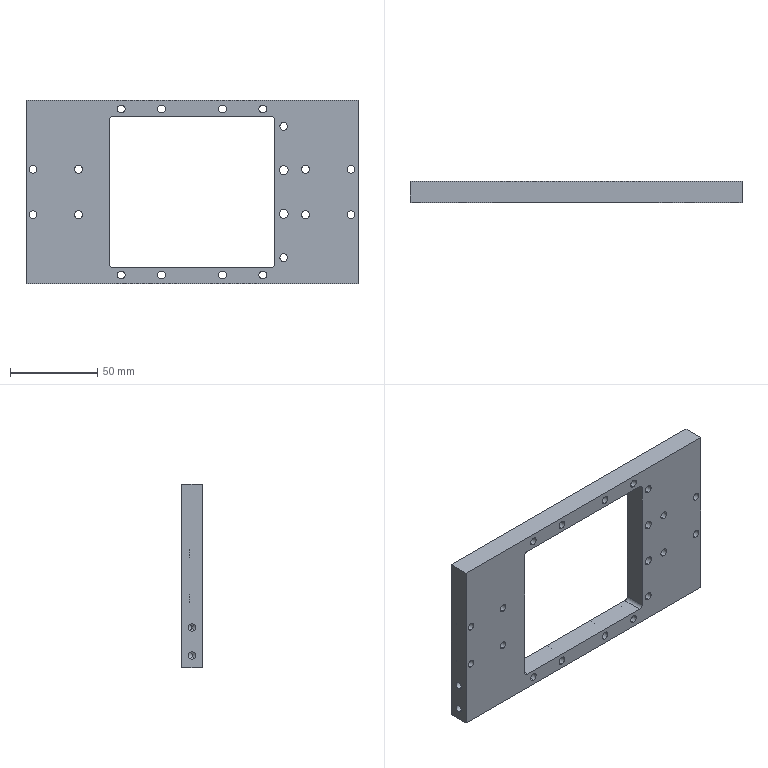Component | SolidWorks | 05-1 | 1 solid | 116 faces | box 190 x 12 x 105 mm | volume 134418 mm3 | cylinder 84 | plane 28 | cone 4 | commonest cylinder face diameters 4.5 x36 8 x20 7.9 x16 4.2 x4 5 x4 4 x4
build123d program:
from build123d import *

# Parameters (mm, degrees)
SKETCH1_W                                       = 190
SKETCH1_H                                       = 105
EXTRUDE1_DEPTH                                  = 6
SKETCH4_W                                       = 95
SKETCH4_H                                       = 86
CUT_EXTRUDE2_DEPTH                              = 110.203
M4_HEX_SOCKET_HEAD_CAP_SCREW_CBORE4_D           = 4.5
M4_HEX_SOCKET_HEAD_CAP_SCREW_CBORE4_CBORE_D     = 7.9
M4_HEX_SOCKET_HEAD_CAP_SCREW_CBORE4_CBORE_DEPTH = 4.4
FILLET1_R                                       = 2
M4_HEX_SOCKET_HEAD_CAP_SCREW_CBORE5_D           = 4.5
M4_HEX_SOCKET_HEAD_CAP_SCREW_CBORE5_CBORE_D     = 8
M4_HEX_SOCKET_HEAD_CAP_SCREW_CBORE5_CBORE_DEPTH = 4.4
SKETCH12_R                                      = 2.5
CUT_EXTRUDE1_DEPTH                              = 35
M5_TAPPED_HOLE1_D                               = 4.2
M5_TAPPED_HOLE1_DEPTH                           = 14
M5_TAPPED_HOLE1_TIP                             = 1.262


with BuildPart() as part:
    # Sketch1 → Extrude1 (new, symmetric)
    with BuildSketch(Plane(origin=(0, 0, 0), x_dir=(1, 0, 0), z_dir=(0, 1, 0))):
        Rectangle(SKETCH1_W, SKETCH1_H)
    extrude(amount=EXTRUDE1_DEPTH, both=True)

    # Sketch4 → Cut-Extrude2 (cut, through all)
    with BuildSketch(Plane(origin=(0, 6, 0), x_dir=(1, 0, 0), z_dir=(0, 1, 0))):
        Rectangle(SKETCH4_W, SKETCH4_H)
    extrude(amount=-CUT_EXTRUDE2_DEPTH, mode=Mode.SUBTRACT)

    # M4 Hex Socket Head Cap Screw CBORE4 (through all)
    with Locations(Plane(origin=(0, 6, 0), x_dir=(1, 0, 0), z_dir=(0, 1, 0))):
        with Locations((91, -13), (65, -13), (91, 13), (65, 13), (-65, -13), (-91, -13), (-65, 13), (-91, 13)):
            CounterBoreHole(M4_HEX_SOCKET_HEAD_CAP_SCREW_CBORE4_D / 2, M4_HEX_SOCKET_HEAD_CAP_SCREW_CBORE4_CBORE_D / 2, M4_HEX_SOCKET_HEAD_CAP_SCREW_CBORE4_CBORE_DEPTH)

    # Fillet1
    fillet1_edges = [part.edges().sort_by_distance(p)[0] for p in [
        (-47.5, 0, 43),
        (-47.5, 0, -43),
        (47.5, 0, -43),
        (47.5, 0, 43),
    ]]
    fillet(fillet1_edges, radius=FILLET1_R)

    # M4 Hex Socket Head Cap Screw CBORE5 (through all)
    with Locations(Plane(origin=(0, 6, 0), x_dir=(1, 0, 0), z_dir=(0, 1, 0))):
        with Locations((40.5, -47.5), (17.5, -47.5), (-17.5, -47.5), (-40.5, -47.5), (40.5, 47.5), (17.5, 47.5), (-17.5, 47.5), (-40.5, 47.5), (52.5, 37.5), (52.5, -37.5)):
            CounterBoreHole(M4_HEX_SOCKET_HEAD_CAP_SCREW_CBORE5_D / 2, M4_HEX_SOCKET_HEAD_CAP_SCREW_CBORE5_CBORE_D / 2, M4_HEX_SOCKET_HEAD_CAP_SCREW_CBORE5_CBORE_DEPTH)

    # Sketch12 → Cut-Extrude1 (cut)
    with BuildSketch(Plane(origin=(0, 6, 0), x_dir=(1, 0, 0), z_dir=(0, 1, 0))):
        with Locations(Location((52.5, -12.5, 0), (0, 0, 270))):
            Circle(SKETCH12_R)
        with Locations(Location((52.5, 12.5, 0), (0, 0, 270))):
            Circle(SKETCH12_R)
    extrude(amount=-CUT_EXTRUDE1_DEPTH, mode=Mode.SUBTRACT)

    # M5 Tapped Hole1
    with Locations(Plane.ZY.offset(95)):
        with Locations((-29.5, 0), (-45.5, 0)):
            Hole(M5_TAPPED_HOLE1_D / 2, depth=M5_TAPPED_HOLE1_DEPTH)
            with Locations((0, 0, -(M5_TAPPED_HOLE1_DEPTH + M5_TAPPED_HOLE1_TIP / 2))):  # 118° drill point
                Cone(0, M5_TAPPED_HOLE1_D / 2, M5_TAPPED_HOLE1_TIP, mode=Mode.SUBTRACT)


solid = part.part

# Placed as in the assembly
solid = solid.moved(Location((8, 22, 139.3), (0, 0, 0)))